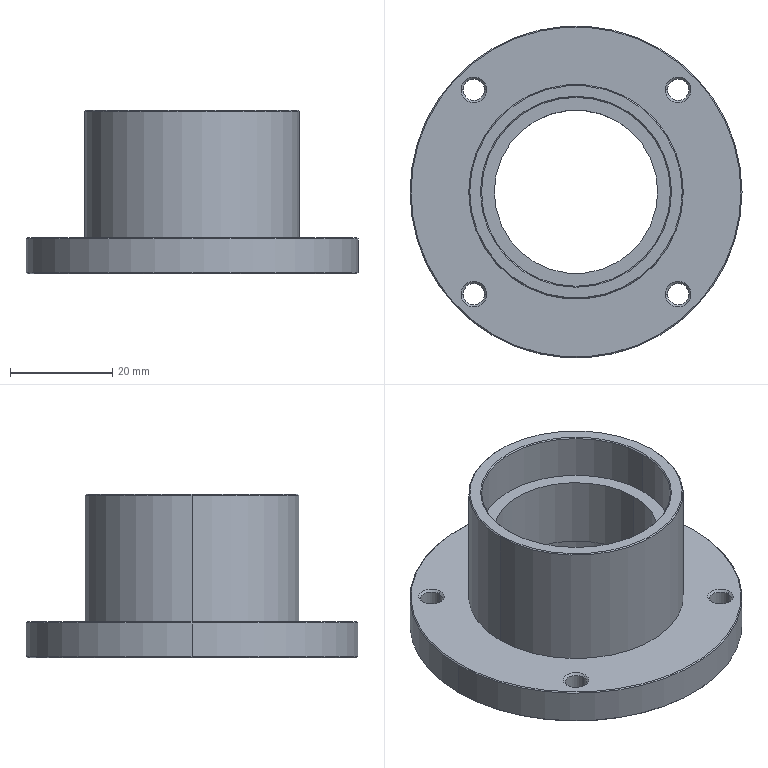Component | SolidWorks | YX-04-104GluePaperFeedingBearingFixingSeat-1 | 1 solid | 41 faces | box 65 x 65 x 32 mm | volume 26843 mm3 | cone 18 | cylinder 18 | plane 5 | commonest cylinder face diameters 4.2 x8 37 x4 32 x2 42 x2 65 x2 | material 45#Steel
build123d program:
from build123d import *

# Parameters (mm, degrees)
SKETCH1_W                  = 7
SKETCH1_H                  = 32.5
SKETCH2_R                  = 21
BOSS_EXTRUDE1_DEPTH        = 25
F_4_2_4_2_DIAMETER_HOLE1_D = 4.2
CHAMFER1_SIZE              = 0.4
CHAMFER2_SIZE              = 0.2


with BuildPart() as part:
    # Sketch1 → Revolve1 (revolve)
    with BuildSketch(Plane.XY, mode=Mode.PRIVATE) as revolve1_sk:
        with Locations((28.5, 16.25)):
            Rectangle(SKETCH1_W, SKETCH1_H)
    revolve(revolve1_sk.sketch.rotate(Axis((25, 0, 0), (1, 0, 0)), 270), axis=Axis((25, 0, 0), (1, 0, 0)))

    # Sketch2 → Boss-Extrude1 (add)
    with BuildSketch(Plane.ZY.offset(-25)):
        Circle(SKETCH2_R)
    extrude(amount=BOSS_EXTRUDE1_DEPTH)

    # Sketch3 → Cut-Revolve1 (revolve, cut)
    with BuildSketch(Plane.XY, mode=Mode.PRIVATE) as cut_revolve1_sk:
        Polygon((0, 18.5), (0, 0), (32, 0), (32, 18.5), (23, 18.5), (23, 16), (9, 16), (9, 18.5), align=None)
    revolve(cut_revolve1_sk.sketch.rotate(Axis((0, 0, 0), (1, 0, 0)), 270), axis=Axis((0, 0, 0), (1, 0, 0)), mode=Mode.SUBTRACT)

    # 4.2 _4.2_ Diameter Hole1 (through all)
    with Locations(Plane.ZY.offset(-25)):
        with Locations((20, -20), (20, 20), (-20, 20), (-20, -20)):
            Hole(F_4_2_4_2_DIAMETER_HOLE1_D / 2)

    # Chamfer1
    chamfer1_edges = [part.edges().sort_by_distance(p)[0] for p in [
        (25, -20, -17.9),
        (25, 20, -17.9),
        (25, 20, 22.1),
        (25, -20, 22.1),
    ]]
    chamfer(chamfer1_edges, length=CHAMFER1_SIZE)

    # Chamfer2
    chamfer2_edges = [part.edges().sort_by_distance(p)[0] for p in [
        (0, 0, -21),
        (0, 0, 18.5),
        (32, 0, 18.5),
        (32, 0, 32.5),
        (25, 0, 32.5),
    ]]
    chamfer(chamfer2_edges, length=CHAMFER2_SIZE)


solid = part.part

# Placed as in the assembly
solid = solid.moved(Location((-103.397, 6.262, 219), (0, 90, 0)))